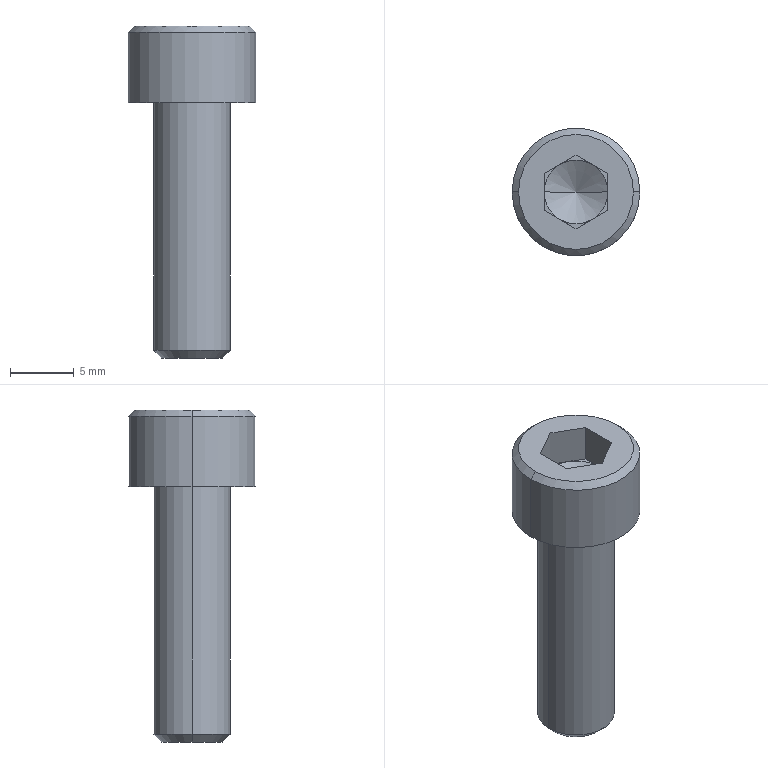Component | SolidWorks | ScrewM6-L20AndSpringWasherAssembly-1_ScrewTAC21-M6-L20(YIHEDA)-1 | 1 solid | 25 faces | box 10 x 10 x 26 mm | volume 955 mm3 | plane 15 | cone 6 | cylinder 4 | commonest cylinder face diameters 10 x2 6 x2
STEP:
#1=CARTESIAN_POINT('',(2.282,0.5813,9.477));
#2=VERTEX_POINT('',#1);
#3=CARTESIAN_POINT('',(2.47,0.5813,9.477));
#4=VERTEX_POINT('',#3);
#5=CARTESIAN_POINT('',(2.376,0.5813,9.477));
#6=DIRECTION('',(0.,0.,-1.));
#7=DIRECTION('',(-1.,0.,0.));
#8=AXIS2_PLACEMENT_3D('',#5,#6,#7);
#9=CIRCLE('',#8,0.09396);
#10=EDGE_CURVE('',#2,#4,#9,.T.);
#11=ORIENTED_EDGE('',*,*,#10,.F.);
#12=CARTESIAN_POINT('',(2.257,0.5813,9.501));
#13=VERTEX_POINT('',#12);
#14=CARTESIAN_POINT('',(2.257,0.5813,9.501));
#15=DIRECTION('',(-0.7071,0.,0.7071));
#16=VECTOR('',#15,39.37);
#17=LINE('',#14,#16);
#18=EDGE_CURVE('',#2,#13,#17,.T.);
#19=ORIENTED_EDGE('',*,*,#18,.T.);
#20=CARTESIAN_POINT('',(2.494,0.5813,9.501));
#21=VERTEX_POINT('',#20);
#22=CARTESIAN_POINT('',(2.376,0.5813,9.501));
#23=DIRECTION('',(0.,0.,-1.));
#24=DIRECTION('',(-1.,0.,0.));
#25=AXIS2_PLACEMENT_3D('',#22,#23,#24);
#26=CIRCLE('',#25,0.1181);
#27=EDGE_CURVE('',#13,#21,#26,.T.);
#28=ORIENTED_EDGE('',*,*,#27,.T.);
#29=CARTESIAN_POINT('',(2.494,0.5813,9.501));
#30=DIRECTION('',(0.7071,0.,0.7071));
#31=VECTOR('',#30,39.37);
#32=LINE('',#29,#31);
#33=EDGE_CURVE('',#4,#21,#32,.T.);
#34=ORIENTED_EDGE('',*,*,#33,.F.);
#35=EDGE_LOOP('',(#11,#19,#28,#34));
#36=FACE_OUTER_BOUND('',#35,.T.);
#37=CARTESIAN_POINT('',(2.376,0.5813,9.501));
#38=DIRECTION('',(0.,0.,1.));
#39=DIRECTION('',(1.,0.,0.));
#40=AXIS2_PLACEMENT_3D('',#37,#38,#39);
#41=CONICAL_SURFACE('',#40,0.1181,0.7854);
#42=ADVANCED_FACE('',(#36),#41,.T.);
#43=CARTESIAN_POINT('',(2.198,0.5813,10.5));
#44=VERTEX_POINT('',#43);
#45=CARTESIAN_POINT('',(2.553,0.5813,10.5));
#46=VERTEX_POINT('',#45);
#47=CARTESIAN_POINT('',(2.376,0.5813,10.5));
#48=DIRECTION('',(0.,0.,-1.));
#49=DIRECTION('',(-1.,0.,0.));
#50=AXIS2_PLACEMENT_3D('',#47,#48,#49);
#51=CIRCLE('',#50,0.1772);
#52=EDGE_CURVE('',#44,#46,#51,.T.);
#53=ORIENTED_EDGE('',*,*,#52,.T.);
#54=CARTESIAN_POINT('',(2.572,0.5813,10.48));
#55=VERTEX_POINT('',#54);
#56=CARTESIAN_POINT('',(2.553,0.5813,10.5));
#57=DIRECTION('',(0.7071,0.,-0.7071));
#58=VECTOR('',#57,39.37);
#59=LINE('',#56,#58);
#60=EDGE_CURVE('',#46,#55,#59,.T.);
#61=ORIENTED_EDGE('',*,*,#60,.T.);
#62=CARTESIAN_POINT('',(2.179,0.5813,10.48));
#63=VERTEX_POINT('',#62);
#64=CARTESIAN_POINT('',(2.376,0.5813,10.48));
#65=DIRECTION('',(0.,0.,-1.));
#66=DIRECTION('',(-1.,0.,0.));
#67=AXIS2_PLACEMENT_3D('',#64,#65,#66);
#68=CIRCLE('',#67,0.1969);
#69=EDGE_CURVE('',#63,#55,#68,.T.);
#70=ORIENTED_EDGE('',*,*,#69,.F.);
#71=CARTESIAN_POINT('',(2.198,0.5813,10.5));
#72=DIRECTION('',(-0.7071,0.,-0.7071));
#73=VECTOR('',#72,39.37);
#74=LINE('',#71,#73);
#75=EDGE_CURVE('',#44,#63,#74,.T.);
#76=ORIENTED_EDGE('',*,*,#75,.F.);
#77=EDGE_LOOP('',(#53,#61,#70,#76));
#78=FACE_OUTER_BOUND('',#77,.T.);
#79=CARTESIAN_POINT('',(2.376,0.5813,10.5));
#80=DIRECTION('',(0.,0.,-1.));
#81=DIRECTION('',(-1.,0.,0.));
#82=AXIS2_PLACEMENT_3D('',#79,#80,#81);
#83=CONICAL_SURFACE('',#82,0.1772,0.7854);
#84=ADVANCED_FACE('',(#78),#83,.T.);
#85=CARTESIAN_POINT('',(2.572,0.5813,10.264));
#86=VERTEX_POINT('',#85);
#87=CARTESIAN_POINT('',(2.179,0.5813,10.264));
#88=VERTEX_POINT('',#87);
#89=CARTESIAN_POINT('',(2.376,0.5813,10.264));
#90=DIRECTION('',(0.,0.,-1.));
#91=DIRECTION('',(-1.,0.,0.));
#92=AXIS2_PLACEMENT_3D('',#89,#90,#91);
#93=CIRCLE('',#92,0.1969);
#94=EDGE_CURVE('',#86,#88,#93,.T.);
#95=ORIENTED_EDGE('',*,*,#94,.F.);
#96=CARTESIAN_POINT('',(2.572,0.5813,10.264));
#97=DIRECTION('',(0.,0.,1.));
#98=VECTOR('',#97,39.37);
#99=LINE('',#96,#98);
#100=EDGE_CURVE('',#86,#55,#99,.T.);
#101=ORIENTED_EDGE('',*,*,#100,.T.);
#102=CARTESIAN_POINT('',(2.376,0.5813,10.48));
#103=DIRECTION('',(0.,0.,-1.));
#104=DIRECTION('',(-1.,0.,0.));
#105=AXIS2_PLACEMENT_3D('',#102,#103,#104);
#106=CIRCLE('',#105,0.1969);
#107=EDGE_CURVE('',#55,#63,#106,.T.);
#108=ORIENTED_EDGE('',*,*,#107,.T.);
#109=CARTESIAN_POINT('',(2.179,0.5813,10.264));
#110=DIRECTION('',(0.,0.,1.));
#111=VECTOR('',#110,39.37);
#112=LINE('',#109,#111);
#113=EDGE_CURVE('',#88,#63,#112,.T.);
#114=ORIENTED_EDGE('',*,*,#113,.F.);
#115=EDGE_LOOP('',(#95,#101,#108,#114));
#116=FACE_OUTER_BOUND('',#115,.T.);
#117=CARTESIAN_POINT('',(2.376,0.5813,10.264));
#118=DIRECTION('',(0.,0.,1.));
#119=DIRECTION('',(-1.,0.,0.));
#120=AXIS2_PLACEMENT_3D('',#117,#118,#119);
#121=CYLINDRICAL_SURFACE('',#120,0.1969);
#122=ADVANCED_FACE('',(#116),#121,.T.);
#123=CARTESIAN_POINT('',(2.376,0.5813,10.325));
#124=VERTEX_POINT('',#123);
#125=CARTESIAN_POINT('',(2.474,0.5813,10.382));
#126=VERTEX_POINT('',#125);
#127=CARTESIAN_POINT('',(2.474,0.5813,10.382));
#128=DIRECTION('',(0.866,0.,0.5));
#129=VECTOR('',#128,39.37);
#130=LINE('',#127,#129);
#131=EDGE_CURVE('',#124,#126,#130,.T.);
#132=ORIENTED_EDGE('',*,*,#131,.F.);
#133=CARTESIAN_POINT('',(2.277,0.5813,10.382));
#134=VERTEX_POINT('',#133);
#135=CARTESIAN_POINT('',(2.277,0.5813,10.382));
#136=DIRECTION('',(-0.866,0.,0.5));
#137=VECTOR('',#136,39.37);
#138=LINE('',#135,#137);
#139=EDGE_CURVE('',#124,#134,#138,.T.);
#140=ORIENTED_EDGE('',*,*,#139,.T.);
#141=CARTESIAN_POINT('',(2.326,0.4961,10.382));
#142=VERTEX_POINT('',#141);
#143=CARTESIAN_POINT('',(2.376,0.5813,10.382));
#144=DIRECTION('',(0.,0.,-1.));
#145=DIRECTION('',(1.,0.,0.));
#146=AXIS2_PLACEMENT_3D('',#143,#144,#145);
#147=CIRCLE('',#146,0.09843);
#148=EDGE_CURVE('',#142,#134,#147,.T.);
#149=ORIENTED_EDGE('',*,*,#148,.F.);
#150=CARTESIAN_POINT('',(2.425,0.4961,10.382));
#151=VERTEX_POINT('',#150);
#152=CARTESIAN_POINT('',(2.376,0.5813,10.382));
#153=DIRECTION('',(0.,0.,-1.));
#154=DIRECTION('',(1.,0.,0.));
#155=AXIS2_PLACEMENT_3D('',#152,#153,#154);
#156=CIRCLE('',#155,0.09843);
#157=EDGE_CURVE('',#151,#142,#156,.T.);
#158=ORIENTED_EDGE('',*,*,#157,.F.);
#159=CARTESIAN_POINT('',(2.376,0.5813,10.382));
#160=DIRECTION('',(0.,0.,-1.));
#161=DIRECTION('',(1.,0.,0.));
#162=AXIS2_PLACEMENT_3D('',#159,#160,#161);
#163=CIRCLE('',#162,0.09843);
#164=EDGE_CURVE('',#126,#151,#163,.T.);
#165=ORIENTED_EDGE('',*,*,#164,.F.);
#166=EDGE_LOOP('',(#132,#140,#149,#158,#165));
#167=FACE_OUTER_BOUND('',#166,.T.);
#168=CARTESIAN_POINT('',(2.376,0.5813,10.382));
#169=DIRECTION('',(0.,0.,1.));
#170=DIRECTION('',(1.,0.,0.));
#171=AXIS2_PLACEMENT_3D('',#168,#169,#170);
#172=CONICAL_SURFACE('',#171,0.09843,1.047);
#173=ADVANCED_FACE('',(#167),#172,.F.);
#174=CARTESIAN_POINT('',(2.376,0.5813,9.501));
#175=DIRECTION('',(0.,0.,-1.));
#176=DIRECTION('',(-1.,0.,0.));
#177=AXIS2_PLACEMENT_3D('',#174,#175,#176);
#178=CIRCLE('',#177,0.1181);
#179=EDGE_CURVE('',#21,#13,#178,.T.);
#180=ORIENTED_EDGE('',*,*,#179,.F.);
#181=CARTESIAN_POINT('',(2.494,0.5813,10.264));
#182=VERTEX_POINT('',#181);
#183=CARTESIAN_POINT('',(2.494,0.5813,9.477));
#184=DIRECTION('',(0.,0.,1.));
#185=VECTOR('',#184,39.37);
#186=LINE('',#183,#185);
#187=EDGE_CURVE('',#21,#182,#186,.T.);
#188=ORIENTED_EDGE('',*,*,#187,.T.);
#189=CARTESIAN_POINT('',(2.257,0.5813,10.264));
#190=VERTEX_POINT('',#189);
#191=CARTESIAN_POINT('',(2.376,0.5813,10.264));
#192=DIRECTION('',(0.,0.,-1.));
#193=DIRECTION('',(-1.,0.,0.));
#194=AXIS2_PLACEMENT_3D('',#191,#192,#193);
#195=CIRCLE('',#194,0.1181);
#196=EDGE_CURVE('',#182,#190,#195,.T.);
#197=ORIENTED_EDGE('',*,*,#196,.T.);
#198=CARTESIAN_POINT('',(2.257,0.5813,9.477));
#199=DIRECTION('',(0.,0.,1.));
#200=VECTOR('',#199,39.37);
#201=LINE('',#198,#200);
#202=EDGE_CURVE('',#13,#190,#201,.T.);
#203=ORIENTED_EDGE('',*,*,#202,.F.);
#204=EDGE_LOOP('',(#180,#188,#197,#203));
#205=FACE_OUTER_BOUND('',#204,.T.);
#206=CARTESIAN_POINT('',(2.376,0.5813,9.477));
#207=DIRECTION('',(0.,0.,1.));
#208=DIRECTION('',(-1.,0.,0.));
#209=AXIS2_PLACEMENT_3D('',#206,#207,#208);
#210=CYLINDRICAL_SURFACE('',#209,0.1181);
#211=ADVANCED_FACE('',(#205),#210,.T.);
#212=CARTESIAN_POINT('',(2.376,0.4677,10.382));
#213=VERTEX_POINT('',#212);
#214=CARTESIAN_POINT('',(2.376,0.4677,10.382));
#215=DIRECTION('',(0.866,0.5,0.));
#216=VECTOR('',#215,39.37);
#217=LINE('',#214,#216);
#218=EDGE_CURVE('',#213,#151,#217,.T.);
#219=ORIENTED_EDGE('',*,*,#218,.T.);
#220=ORIENTED_EDGE('',*,*,#157,.T.);
#221=CARTESIAN_POINT('',(2.277,0.5245,10.382));
#222=DIRECTION('',(0.866,-0.5,0.));
#223=VECTOR('',#222,39.37);
#224=LINE('',#221,#223);
#225=EDGE_CURVE('',#142,#213,#224,.T.);
#226=ORIENTED_EDGE('',*,*,#225,.T.);
#227=EDGE_LOOP('',(#219,#220,#226));
#228=FACE_OUTER_BOUND('',#227,.T.);
#229=CARTESIAN_POINT('',(2.376,0.5813,10.382));
#230=DIRECTION('',(0.,0.,1.));
#231=DIRECTION('',(1.,0.,0.));
#232=AXIS2_PLACEMENT_3D('',#229,#230,#231);
#233=PLANE('',#232);
#234=ADVANCED_FACE('',(#228),#233,.T.);
#235=ORIENTED_EDGE('',*,*,#187,.F.);
#236=ORIENTED_EDGE('',*,*,#27,.F.);
#237=ORIENTED_EDGE('',*,*,#202,.T.);
#238=CARTESIAN_POINT('',(2.376,0.5813,10.264));
#239=DIRECTION('',(0.,0.,-1.));
#240=DIRECTION('',(-1.,0.,0.));
#241=AXIS2_PLACEMENT_3D('',#238,#239,#240);
#242=CIRCLE('',#241,0.1181);
#243=EDGE_CURVE('',#190,#182,#242,.T.);
#244=ORIENTED_EDGE('',*,*,#243,.T.);
#245=EDGE_LOOP('',(#235,#236,#237,#244));
#246=FACE_OUTER_BOUND('',#245,.T.);
#247=CARTESIAN_POINT('',(2.376,0.5813,9.477));
#248=DIRECTION('',(0.,0.,1.));
#249=DIRECTION('',(-1.,0.,0.));
#250=AXIS2_PLACEMENT_3D('',#247,#248,#249);
#251=CYLINDRICAL_SURFACE('',#250,0.1181);
#252=ADVANCED_FACE('',(#246),#251,.T.);
#253=ORIENTED_EDGE('',*,*,#139,.F.);
#254=ORIENTED_EDGE('',*,*,#131,.T.);
#255=CARTESIAN_POINT('',(2.425,0.6666,10.382));
#256=VERTEX_POINT('',#255);
#257=CARTESIAN_POINT('',(2.376,0.5813,10.382));
#258=DIRECTION('',(0.,0.,-1.));
#259=DIRECTION('',(1.,0.,0.));
#260=AXIS2_PLACEMENT_3D('',#257,#258,#259);
#261=CIRCLE('',#260,0.09843);
#262=EDGE_CURVE('',#256,#126,#261,.T.);
#263=ORIENTED_EDGE('',*,*,#262,.F.);
#264=CARTESIAN_POINT('',(2.326,0.6666,10.382));
#265=VERTEX_POINT('',#264);
#266=CARTESIAN_POINT('',(2.376,0.5813,10.382));
#267=DIRECTION('',(0.,0.,-1.));
#268=DIRECTION('',(1.,0.,0.));
#269=AXIS2_PLACEMENT_3D('',#266,#267,#268);
#270=CIRCLE('',#269,0.09843);
#271=EDGE_CURVE('',#265,#256,#270,.T.);
#272=ORIENTED_EDGE('',*,*,#271,.F.);
#273=CARTESIAN_POINT('',(2.376,0.5813,10.382));
#274=DIRECTION('',(0.,0.,-1.));
#275=DIRECTION('',(1.,0.,0.));
#276=AXIS2_PLACEMENT_3D('',#273,#274,#275);
#277=CIRCLE('',#276,0.09843);
#278=EDGE_CURVE('',#134,#265,#277,.T.);
#279=ORIENTED_EDGE('',*,*,#278,.F.);
#280=EDGE_LOOP('',(#253,#254,#263,#272,#279));
#281=FACE_OUTER_BOUND('',#280,.T.);
#282=CARTESIAN_POINT('',(2.376,0.5813,10.382));
#283=DIRECTION('',(0.,0.,1.));
#284=DIRECTION('',(1.,0.,0.));
#285=AXIS2_PLACEMENT_3D('',#282,#283,#284);
#286=CONICAL_SURFACE('',#285,0.09843,1.047);
#287=ADVANCED_FACE('',(#281),#286,.F.);
#288=CARTESIAN_POINT('',(2.277,0.6382,10.5));
#289=VERTEX_POINT('',#288);
#290=CARTESIAN_POINT('',(2.277,0.5245,10.5));
#291=VERTEX_POINT('',#290);
#292=CARTESIAN_POINT('',(2.277,0.6382,10.5));
#293=DIRECTION('',(0.,-1.,0.));
#294=VECTOR('',#293,39.37);
#295=LINE('',#292,#294);
#296=EDGE_CURVE('',#289,#291,#295,.T.);
#297=ORIENTED_EDGE('',*,*,#296,.T.);
#298=CARTESIAN_POINT('',(2.277,0.5245,10.382));
#299=VERTEX_POINT('',#298);
#300=CARTESIAN_POINT('',(2.277,0.5245,10.382));
#301=DIRECTION('',(0.,0.,1.));
#302=VECTOR('',#301,39.37);
#303=LINE('',#300,#302);
#304=EDGE_CURVE('',#299,#291,#303,.T.);
#305=ORIENTED_EDGE('',*,*,#304,.F.);
#306=CARTESIAN_POINT('',(2.277,0.6382,10.382));
#307=DIRECTION('',(0.,-1.,0.));
#308=VECTOR('',#307,39.37);
#309=LINE('',#306,#308);
#310=EDGE_CURVE('',#134,#299,#309,.T.);
#311=ORIENTED_EDGE('',*,*,#310,.F.);
#312=CARTESIAN_POINT('',(2.277,0.6382,10.382));
#313=VERTEX_POINT('',#312);
#314=CARTESIAN_POINT('',(2.277,0.6382,10.382));
#315=DIRECTION('',(0.,-1.,0.));
#316=VECTOR('',#315,39.37);
#317=LINE('',#314,#316);
#318=EDGE_CURVE('',#313,#134,#317,.T.);
#319=ORIENTED_EDGE('',*,*,#318,.F.);
#320=CARTESIAN_POINT('',(2.277,0.6382,10.382));
#321=DIRECTION('',(0.,0.,1.));
#322=VECTOR('',#321,39.37);
#323=LINE('',#320,#322);
#324=EDGE_CURVE('',#313,#289,#323,.T.);
#325=ORIENTED_EDGE('',*,*,#324,.T.);
#326=EDGE_LOOP('',(#297,#305,#311,#319,#325));
#327=FACE_OUTER_BOUND('',#326,.T.);
#328=CARTESIAN_POINT('',(2.277,0.6382,10.382));
#329=DIRECTION('',(-1.,0.,0.));
#330=DIRECTION('',(0.,0.,1.));
#331=AXIS2_PLACEMENT_3D('',#328,#329,#330);
#332=PLANE('',#331);
#333=ADVANCED_FACE('',(#327),#332,.F.);
#334=CARTESIAN_POINT('',(2.474,0.6382,10.5));
#335=VERTEX_POINT('',#334);
#336=CARTESIAN_POINT('',(2.376,0.695,10.5));
#337=VERTEX_POINT('',#336);
#338=CARTESIAN_POINT('',(2.474,0.6382,10.5));
#339=DIRECTION('',(-0.866,0.5,0.));
#340=VECTOR('',#339,39.37);
#341=LINE('',#338,#340);
#342=EDGE_CURVE('',#335,#337,#341,.T.);
#343=ORIENTED_EDGE('',*,*,#342,.T.);
#344=CARTESIAN_POINT('',(2.376,0.695,10.382));
#345=VERTEX_POINT('',#344);
#346=CARTESIAN_POINT('',(2.376,0.695,10.382));
#347=DIRECTION('',(0.,0.,1.));
#348=VECTOR('',#347,39.37);
#349=LINE('',#346,#348);
#350=EDGE_CURVE('',#345,#337,#349,.T.);
#351=ORIENTED_EDGE('',*,*,#350,.F.);
#352=CARTESIAN_POINT('',(2.474,0.6382,10.382));
#353=DIRECTION('',(-0.866,0.5,0.));
#354=VECTOR('',#353,39.37);
#355=LINE('',#352,#354);
#356=EDGE_CURVE('',#256,#345,#355,.T.);
#357=ORIENTED_EDGE('',*,*,#356,.F.);
#358=CARTESIAN_POINT('',(2.474,0.6382,10.382));
#359=VERTEX_POINT('',#358);
#360=CARTESIAN_POINT('',(2.474,0.6382,10.382));
#361=DIRECTION('',(-0.866,0.5,0.));
#362=VECTOR('',#361,39.37);
#363=LINE('',#360,#362);
#364=EDGE_CURVE('',#359,#256,#363,.T.);
#365=ORIENTED_EDGE('',*,*,#364,.F.);
#366=CARTESIAN_POINT('',(2.474,0.6382,10.382));
#367=DIRECTION('',(0.,0.,1.));
#368=VECTOR('',#367,39.37);
#369=LINE('',#366,#368);
#370=EDGE_CURVE('',#359,#335,#369,.T.);
#371=ORIENTED_EDGE('',*,*,#370,.T.);
#372=EDGE_LOOP('',(#343,#351,#357,#365,#371));
#373=FACE_OUTER_BOUND('',#372,.T.);
#374=CARTESIAN_POINT('',(2.474,0.6382,10.382));
#375=DIRECTION('',(0.5,0.866,0.));
#376=DIRECTION('',(0.,0.,-1.));
#377=AXIS2_PLACEMENT_3D('',#374,#375,#376);
#378=PLANE('',#377);
#379=ADVANCED_FACE('',(#373),#378,.F.);
#380=ORIENTED_EDGE('',*,*,#364,.T.);
#381=ORIENTED_EDGE('',*,*,#262,.T.);
#382=CARTESIAN_POINT('',(2.474,0.5245,10.382));
#383=DIRECTION('',(0.,1.,0.));
#384=VECTOR('',#383,39.37);
#385=LINE('',#382,#384);
#386=EDGE_CURVE('',#126,#359,#385,.T.);
#387=ORIENTED_EDGE('',*,*,#386,.T.);
#388=EDGE_LOOP('',(#380,#381,#387));
#389=FACE_OUTER_BOUND('',#388,.T.);
#390=CARTESIAN_POINT('',(2.376,0.5813,10.382));
#391=DIRECTION('',(0.,0.,1.));
#392=DIRECTION('',(1.,0.,0.));
#393=AXIS2_PLACEMENT_3D('',#390,#391,#392);
#394=PLANE('',#393);
#395=ADVANCED_FACE('',(#389),#394,.T.);
#396=CARTESIAN_POINT('',(2.376,0.5813,10.264));
#397=DIRECTION('',(0.,0.,-1.));
#398=DIRECTION('',(-1.,0.,0.));
#399=AXIS2_PLACEMENT_3D('',#396,#397,#398);
#400=CIRCLE('',#399,0.1969);
#401=EDGE_CURVE('',#88,#86,#400,.T.);
#402=ORIENTED_EDGE('',*,*,#401,.T.);
#403=ORIENTED_EDGE('',*,*,#94,.T.);
#404=EDGE_LOOP('',(#402,#403));
#405=FACE_OUTER_BOUND('',#404,.T.);
#406=ORIENTED_EDGE('',*,*,#243,.F.);
#407=ORIENTED_EDGE('',*,*,#196,.F.);
#408=EDGE_LOOP('',(#406,#407));
#409=FACE_BOUND('',#408,.T.);
#410=CARTESIAN_POINT('',(2.376,0.7782,10.264));
#411=DIRECTION('',(0.,0.,1.));
#412=DIRECTION('',(1.,0.,0.));
#413=AXIS2_PLACEMENT_3D('',#410,#411,#412);
#414=PLANE('',#413);
#415=ADVANCED_FACE('',(#405,#409),#414,.F.);
#416=ORIENTED_EDGE('',*,*,#52,.F.);
#417=CARTESIAN_POINT('',(2.376,0.5813,10.5));
#418=DIRECTION('',(0.,0.,-1.));
#419=DIRECTION('',(-1.,0.,0.));
#420=AXIS2_PLACEMENT_3D('',#417,#418,#419);
#421=CIRCLE('',#420,0.1772);
#422=EDGE_CURVE('',#46,#44,#421,.T.);
#423=ORIENTED_EDGE('',*,*,#422,.F.);
#424=EDGE_LOOP('',(#416,#423));
#425=FACE_OUTER_BOUND('',#424,.T.);
#426=CARTESIAN_POINT('',(2.376,0.4677,10.5));
#427=VERTEX_POINT('',#426);
#428=CARTESIAN_POINT('',(2.474,0.5245,10.5));
#429=VERTEX_POINT('',#428);
#430=CARTESIAN_POINT('',(2.376,0.4677,10.5));
#431=DIRECTION('',(0.866,0.5,0.));
#432=VECTOR('',#431,39.37);
#433=LINE('',#430,#432);
#434=EDGE_CURVE('',#427,#429,#433,.T.);
#435=ORIENTED_EDGE('',*,*,#434,.F.);
#436=CARTESIAN_POINT('',(2.277,0.5245,10.5));
#437=DIRECTION('',(0.866,-0.5,0.));
#438=VECTOR('',#437,39.37);
#439=LINE('',#436,#438);
#440=EDGE_CURVE('',#291,#427,#439,.T.);
#441=ORIENTED_EDGE('',*,*,#440,.F.);
#442=ORIENTED_EDGE('',*,*,#296,.F.);
#443=CARTESIAN_POINT('',(2.376,0.695,10.5));
#444=DIRECTION('',(-0.866,-0.5,0.));
#445=VECTOR('',#444,39.37);
#446=LINE('',#443,#445);
#447=EDGE_CURVE('',#337,#289,#446,.T.);
#448=ORIENTED_EDGE('',*,*,#447,.F.);
#449=ORIENTED_EDGE('',*,*,#342,.F.);
#450=CARTESIAN_POINT('',(2.474,0.5245,10.5));
#451=DIRECTION('',(0.,1.,0.));
#452=VECTOR('',#451,39.37);
#453=LINE('',#450,#452);
#454=EDGE_CURVE('',#429,#335,#453,.T.);
#455=ORIENTED_EDGE('',*,*,#454,.F.);
#456=EDGE_LOOP('',(#435,#441,#442,#448,#449,#455));
#457=FACE_BOUND('',#456,.T.);
#458=CARTESIAN_POINT('',(2.376,0.5813,10.5));
#459=DIRECTION('',(0.,0.,-1.));
#460=DIRECTION('',(0.,-1.,0.));
#461=AXIS2_PLACEMENT_3D('',#458,#459,#460);
#462=PLANE('',#461);
#463=ADVANCED_FACE('',(#425,#457),#462,.F.);
#464=CARTESIAN_POINT('',(2.376,0.5813,9.477));
#465=DIRECTION('',(0.,0.,-1.));
#466=DIRECTION('',(-1.,0.,0.));
#467=AXIS2_PLACEMENT_3D('',#464,#465,#466);
#468=CIRCLE('',#467,0.09396);
#469=EDGE_CURVE('',#4,#2,#468,.T.);
#470=ORIENTED_EDGE('',*,*,#469,.T.);
#471=ORIENTED_EDGE('',*,*,#10,.T.);
#472=EDGE_LOOP('',(#470,#471));
#473=FACE_OUTER_BOUND('',#472,.T.);
#474=CARTESIAN_POINT('',(2.376,0.6753,9.477));
#475=DIRECTION('',(0.,0.,1.));
#476=DIRECTION('',(1.,0.,0.));
#477=AXIS2_PLACEMENT_3D('',#474,#475,#476);
#478=PLANE('',#477);
#479=ADVANCED_FACE('',(#473),#478,.F.);
#480=ORIENTED_EDGE('',*,*,#100,.F.);
#481=ORIENTED_EDGE('',*,*,#401,.F.);
#482=ORIENTED_EDGE('',*,*,#113,.T.);
#483=ORIENTED_EDGE('',*,*,#69,.T.);
#484=EDGE_LOOP('',(#480,#481,#482,#483));
#485=FACE_OUTER_BOUND('',#484,.T.);
#486=CARTESIAN_POINT('',(2.376,0.5813,10.264));
#487=DIRECTION('',(0.,0.,1.));
#488=DIRECTION('',(-1.,0.,0.));
#489=AXIS2_PLACEMENT_3D('',#486,#487,#488);
#490=CYLINDRICAL_SURFACE('',#489,0.1969);
#491=ADVANCED_FACE('',(#485),#490,.T.);
#492=ORIENTED_EDGE('',*,*,#440,.T.);
#493=CARTESIAN_POINT('',(2.376,0.4677,10.382));
#494=DIRECTION('',(0.,0.,1.));
#495=VECTOR('',#494,39.37);
#496=LINE('',#493,#495);
#497=EDGE_CURVE('',#213,#427,#496,.T.);
#498=ORIENTED_EDGE('',*,*,#497,.F.);
#499=ORIENTED_EDGE('',*,*,#225,.F.);
#500=CARTESIAN_POINT('',(2.277,0.5245,10.382));
#501=DIRECTION('',(0.866,-0.5,0.));
#502=VECTOR('',#501,39.37);
#503=LINE('',#500,#502);
#504=EDGE_CURVE('',#299,#142,#503,.T.);
#505=ORIENTED_EDGE('',*,*,#504,.F.);
#506=ORIENTED_EDGE('',*,*,#304,.T.);
#507=EDGE_LOOP('',(#492,#498,#499,#505,#506));
#508=FACE_OUTER_BOUND('',#507,.T.);
#509=CARTESIAN_POINT('',(2.277,0.5245,10.382));
#510=DIRECTION('',(-0.5,-0.866,0.));
#511=DIRECTION('',(-0.866,0.5,0.));
#512=AXIS2_PLACEMENT_3D('',#509,#510,#511);
#513=PLANE('',#512);
#514=ADVANCED_FACE('',(#508),#513,.F.);
#515=ORIENTED_EDGE('',*,*,#60,.F.);
#516=ORIENTED_EDGE('',*,*,#422,.T.);
#517=ORIENTED_EDGE('',*,*,#75,.T.);
#518=ORIENTED_EDGE('',*,*,#107,.F.);
#519=EDGE_LOOP('',(#515,#516,#517,#518));
#520=FACE_OUTER_BOUND('',#519,.T.);
#521=CARTESIAN_POINT('',(2.376,0.5813,10.5));
#522=DIRECTION('',(0.,0.,-1.));
#523=DIRECTION('',(-1.,0.,0.));
#524=AXIS2_PLACEMENT_3D('',#521,#522,#523);
#525=CONICAL_SURFACE('',#524,0.1772,0.7854);
#526=ADVANCED_FACE('',(#520),#525,.T.);
#527=ORIENTED_EDGE('',*,*,#434,.T.);
#528=CARTESIAN_POINT('',(2.474,0.5245,10.382));
#529=VERTEX_POINT('',#528);
#530=CARTESIAN_POINT('',(2.474,0.5245,10.382));
#531=DIRECTION('',(0.,0.,1.));
#532=VECTOR('',#531,39.37);
#533=LINE('',#530,#532);
#534=EDGE_CURVE('',#529,#429,#533,.T.);
#535=ORIENTED_EDGE('',*,*,#534,.F.);
#536=CARTESIAN_POINT('',(2.376,0.4677,10.382));
#537=DIRECTION('',(0.866,0.5,0.));
#538=VECTOR('',#537,39.37);
#539=LINE('',#536,#538);
#540=EDGE_CURVE('',#151,#529,#539,.T.);
#541=ORIENTED_EDGE('',*,*,#540,.F.);
#542=ORIENTED_EDGE('',*,*,#218,.F.);
#543=ORIENTED_EDGE('',*,*,#497,.T.);
#544=EDGE_LOOP('',(#527,#535,#541,#542,#543));
#545=FACE_OUTER_BOUND('',#544,.T.);
#546=CARTESIAN_POINT('',(2.376,0.4677,10.382));
#547=DIRECTION('',(0.5,-0.866,0.));
#548=DIRECTION('',(0.,0.,-1.));
#549=AXIS2_PLACEMENT_3D('',#546,#547,#548);
#550=PLANE('',#549);
#551=ADVANCED_FACE('',(#545),#550,.F.);
#552=ORIENTED_EDGE('',*,*,#454,.T.);
#553=ORIENTED_EDGE('',*,*,#370,.F.);
#554=ORIENTED_EDGE('',*,*,#386,.F.);
#555=CARTESIAN_POINT('',(2.474,0.5245,10.382));
#556=DIRECTION('',(0.,1.,0.));
#557=VECTOR('',#556,39.37);
#558=LINE('',#555,#557);
#559=EDGE_CURVE('',#529,#126,#558,.T.);
#560=ORIENTED_EDGE('',*,*,#559,.F.);
#561=ORIENTED_EDGE('',*,*,#534,.T.);
#562=EDGE_LOOP('',(#552,#553,#554,#560,#561));
#563=FACE_OUTER_BOUND('',#562,.T.);
#564=CARTESIAN_POINT('',(2.474,0.5245,10.382));
#565=DIRECTION('',(1.,0.,0.));
#566=DIRECTION('',(0.,1.,0.));
#567=AXIS2_PLACEMENT_3D('',#564,#565,#566);
#568=PLANE('',#567);
#569=ADVANCED_FACE('',(#563),#568,.F.);
#570=ORIENTED_EDGE('',*,*,#559,.T.);
#571=ORIENTED_EDGE('',*,*,#164,.T.);
#572=ORIENTED_EDGE('',*,*,#540,.T.);
#573=EDGE_LOOP('',(#570,#571,#572));
#574=FACE_OUTER_BOUND('',#573,.T.);
#575=CARTESIAN_POINT('',(2.376,0.5813,10.382));
#576=DIRECTION('',(0.,0.,1.));
#577=DIRECTION('',(1.,0.,0.));
#578=AXIS2_PLACEMENT_3D('',#575,#576,#577);
#579=PLANE('',#578);
#580=ADVANCED_FACE('',(#574),#579,.T.);
#581=ORIENTED_EDGE('',*,*,#504,.T.);
#582=ORIENTED_EDGE('',*,*,#148,.T.);
#583=ORIENTED_EDGE('',*,*,#310,.T.);
#584=EDGE_LOOP('',(#581,#582,#583));
#585=FACE_OUTER_BOUND('',#584,.T.);
#586=CARTESIAN_POINT('',(2.376,0.5813,10.382));
#587=DIRECTION('',(0.,0.,1.));
#588=DIRECTION('',(1.,0.,0.));
#589=AXIS2_PLACEMENT_3D('',#586,#587,#588);
#590=PLANE('',#589);
#591=ADVANCED_FACE('',(#585),#590,.T.);
#592=ORIENTED_EDGE('',*,*,#318,.T.);
#593=ORIENTED_EDGE('',*,*,#278,.T.);
#594=CARTESIAN_POINT('',(2.376,0.695,10.382));
#595=DIRECTION('',(-0.866,-0.5,0.));
#596=VECTOR('',#595,39.37);
#597=LINE('',#594,#596);
#598=EDGE_CURVE('',#265,#313,#597,.T.);
#599=ORIENTED_EDGE('',*,*,#598,.T.);
#600=EDGE_LOOP('',(#592,#593,#599));
#601=FACE_OUTER_BOUND('',#600,.T.);
#602=CARTESIAN_POINT('',(2.376,0.5813,10.382));
#603=DIRECTION('',(0.,0.,1.));
#604=DIRECTION('',(1.,0.,0.));
#605=AXIS2_PLACEMENT_3D('',#602,#603,#604);
#606=PLANE('',#605);
#607=ADVANCED_FACE('',(#601),#606,.T.);
#608=ORIENTED_EDGE('',*,*,#447,.T.);
#609=ORIENTED_EDGE('',*,*,#324,.F.);
#610=ORIENTED_EDGE('',*,*,#598,.F.);
#611=CARTESIAN_POINT('',(2.376,0.695,10.382));
#612=DIRECTION('',(-0.866,-0.5,0.));
#613=VECTOR('',#612,39.37);
#614=LINE('',#611,#613);
#615=EDGE_CURVE('',#345,#265,#614,.T.);
#616=ORIENTED_EDGE('',*,*,#615,.F.);
#617=ORIENTED_EDGE('',*,*,#350,.T.);
#618=EDGE_LOOP('',(#608,#609,#610,#616,#617));
#619=FACE_OUTER_BOUND('',#618,.T.);
#620=CARTESIAN_POINT('',(2.376,0.695,10.382));
#621=DIRECTION('',(-0.5,0.866,0.));
#622=DIRECTION('',(0.,0.,1.));
#623=AXIS2_PLACEMENT_3D('',#620,#621,#622);
#624=PLANE('',#623);
#625=ADVANCED_FACE('',(#619),#624,.F.);
#626=ORIENTED_EDGE('',*,*,#18,.F.);
#627=ORIENTED_EDGE('',*,*,#469,.F.);
#628=ORIENTED_EDGE('',*,*,#33,.T.);
#629=ORIENTED_EDGE('',*,*,#179,.T.);
#630=EDGE_LOOP('',(#626,#627,#628,#629));
#631=FACE_OUTER_BOUND('',#630,.T.);
#632=CARTESIAN_POINT('',(2.376,0.5813,9.501));
#633=DIRECTION('',(0.,0.,1.));
#634=DIRECTION('',(1.,0.,0.));
#635=AXIS2_PLACEMENT_3D('',#632,#633,#634);
#636=CONICAL_SURFACE('',#635,0.1181,0.7854);
#637=ADVANCED_FACE('',(#631),#636,.T.);
#638=ORIENTED_EDGE('',*,*,#615,.T.);
#639=ORIENTED_EDGE('',*,*,#271,.T.);
#640=ORIENTED_EDGE('',*,*,#356,.T.);
#641=EDGE_LOOP('',(#638,#639,#640));
#642=FACE_OUTER_BOUND('',#641,.T.);
#643=CARTESIAN_POINT('',(2.376,0.5813,10.382));
#644=DIRECTION('',(0.,0.,1.));
#645=DIRECTION('',(1.,0.,0.));
#646=AXIS2_PLACEMENT_3D('',#643,#644,#645);
#647=PLANE('',#646);
#648=ADVANCED_FACE('',(#642),#647,.T.);
#649=CLOSED_SHELL('',(#42,#84,#122,#173,#211,#234,#252,#287,#333,#379,#395,#415,#463,#479,#491,#514,#526,#551,#569,#580,#591,#607,#625,#637,#648));
#650=MANIFOLD_SOLID_BREP('',#649);
#651=CARTESIAN_POINT('',(0.,0.,0.));
#652=DIRECTION('',(0.,0.,1.));
#653=DIRECTION('',(1.,0.,0.));
#654=AXIS2_PLACEMENT_3D('',#651,#652,#653);
#655=(LENGTH_UNIT()NAMED_UNIT(*)SI_UNIT($,.METRE.));
#656=LENGTH_MEASURE_WITH_UNIT(LENGTH_MEASURE(0.0254),#655);
#657=DIMENSIONAL_EXPONENTS(1.,0.,0.,0.,0.,0.,0.);
#658=(CONVERSION_BASED_UNIT('',#656)LENGTH_UNIT()NAMED_UNIT(#657));
#659=UNCERTAINTY_MEASURE_WITH_UNIT(LENGTH_MEASURE(0.00001),#658,'','');
#660=(NAMED_UNIT(*)PLANE_ANGLE_UNIT()SI_UNIT($,.RADIAN.));
#661=(NAMED_UNIT(*)SI_UNIT($,.STERADIAN.)SOLID_ANGLE_UNIT());
#662=(GEOMETRIC_REPRESENTATION_CONTEXT(3)GLOBAL_UNCERTAINTY_ASSIGNED_CONTEXT((#659))GLOBAL_UNIT_ASSIGNED_CONTEXT((#658,#660,#661))REPRESENTATION_CONTEXT('',''));
#663=ADVANCED_BREP_SHAPE_REPRESENTATION('',(#650,#654),#662);
#664=COLOUR_RGB('',0.7922,0.8196,0.9333);
#665=FILL_AREA_STYLE_COLOUR('',#664);
#666=FILL_AREA_STYLE('',(#665));
#667=SURFACE_STYLE_FILL_AREA(#666);
#668=SURFACE_SIDE_STYLE('',(#667));
#669=SURFACE_STYLE_USAGE(.BOTH.,#668);
#670=PRESENTATION_STYLE_ASSIGNMENT((#669));
#671=STYLED_ITEM('',(#670),#650);
#672=(LENGTH_UNIT()NAMED_UNIT(*)SI_UNIT($,.METRE.));
#673=LENGTH_MEASURE_WITH_UNIT(LENGTH_MEASURE(0.0254),#672);
#674=DIMENSIONAL_EXPONENTS(1.,0.,0.,0.,0.,0.,0.);
#675=(CONVERSION_BASED_UNIT('',#673)LENGTH_UNIT()NAMED_UNIT(#674));
#676=UNCERTAINTY_MEASURE_WITH_UNIT(LENGTH_MEASURE(0.00001),#675,'','');
#677=(NAMED_UNIT(*)PLANE_ANGLE_UNIT()SI_UNIT($,.RADIAN.));
#678=(NAMED_UNIT(*)SI_UNIT($,.STERADIAN.)SOLID_ANGLE_UNIT());
#679=(GEOMETRIC_REPRESENTATION_CONTEXT(3)GLOBAL_UNCERTAINTY_ASSIGNED_CONTEXT((#676))GLOBAL_UNIT_ASSIGNED_CONTEXT((#675,#677,#678))REPRESENTATION_CONTEXT('',''));
#680=MECHANICAL_DESIGN_GEOMETRIC_PRESENTATION_REPRESENTATION('',(#671),#679);
#681=PRESENTATION_LAYER_ASSIGNMENT('','',(#671));